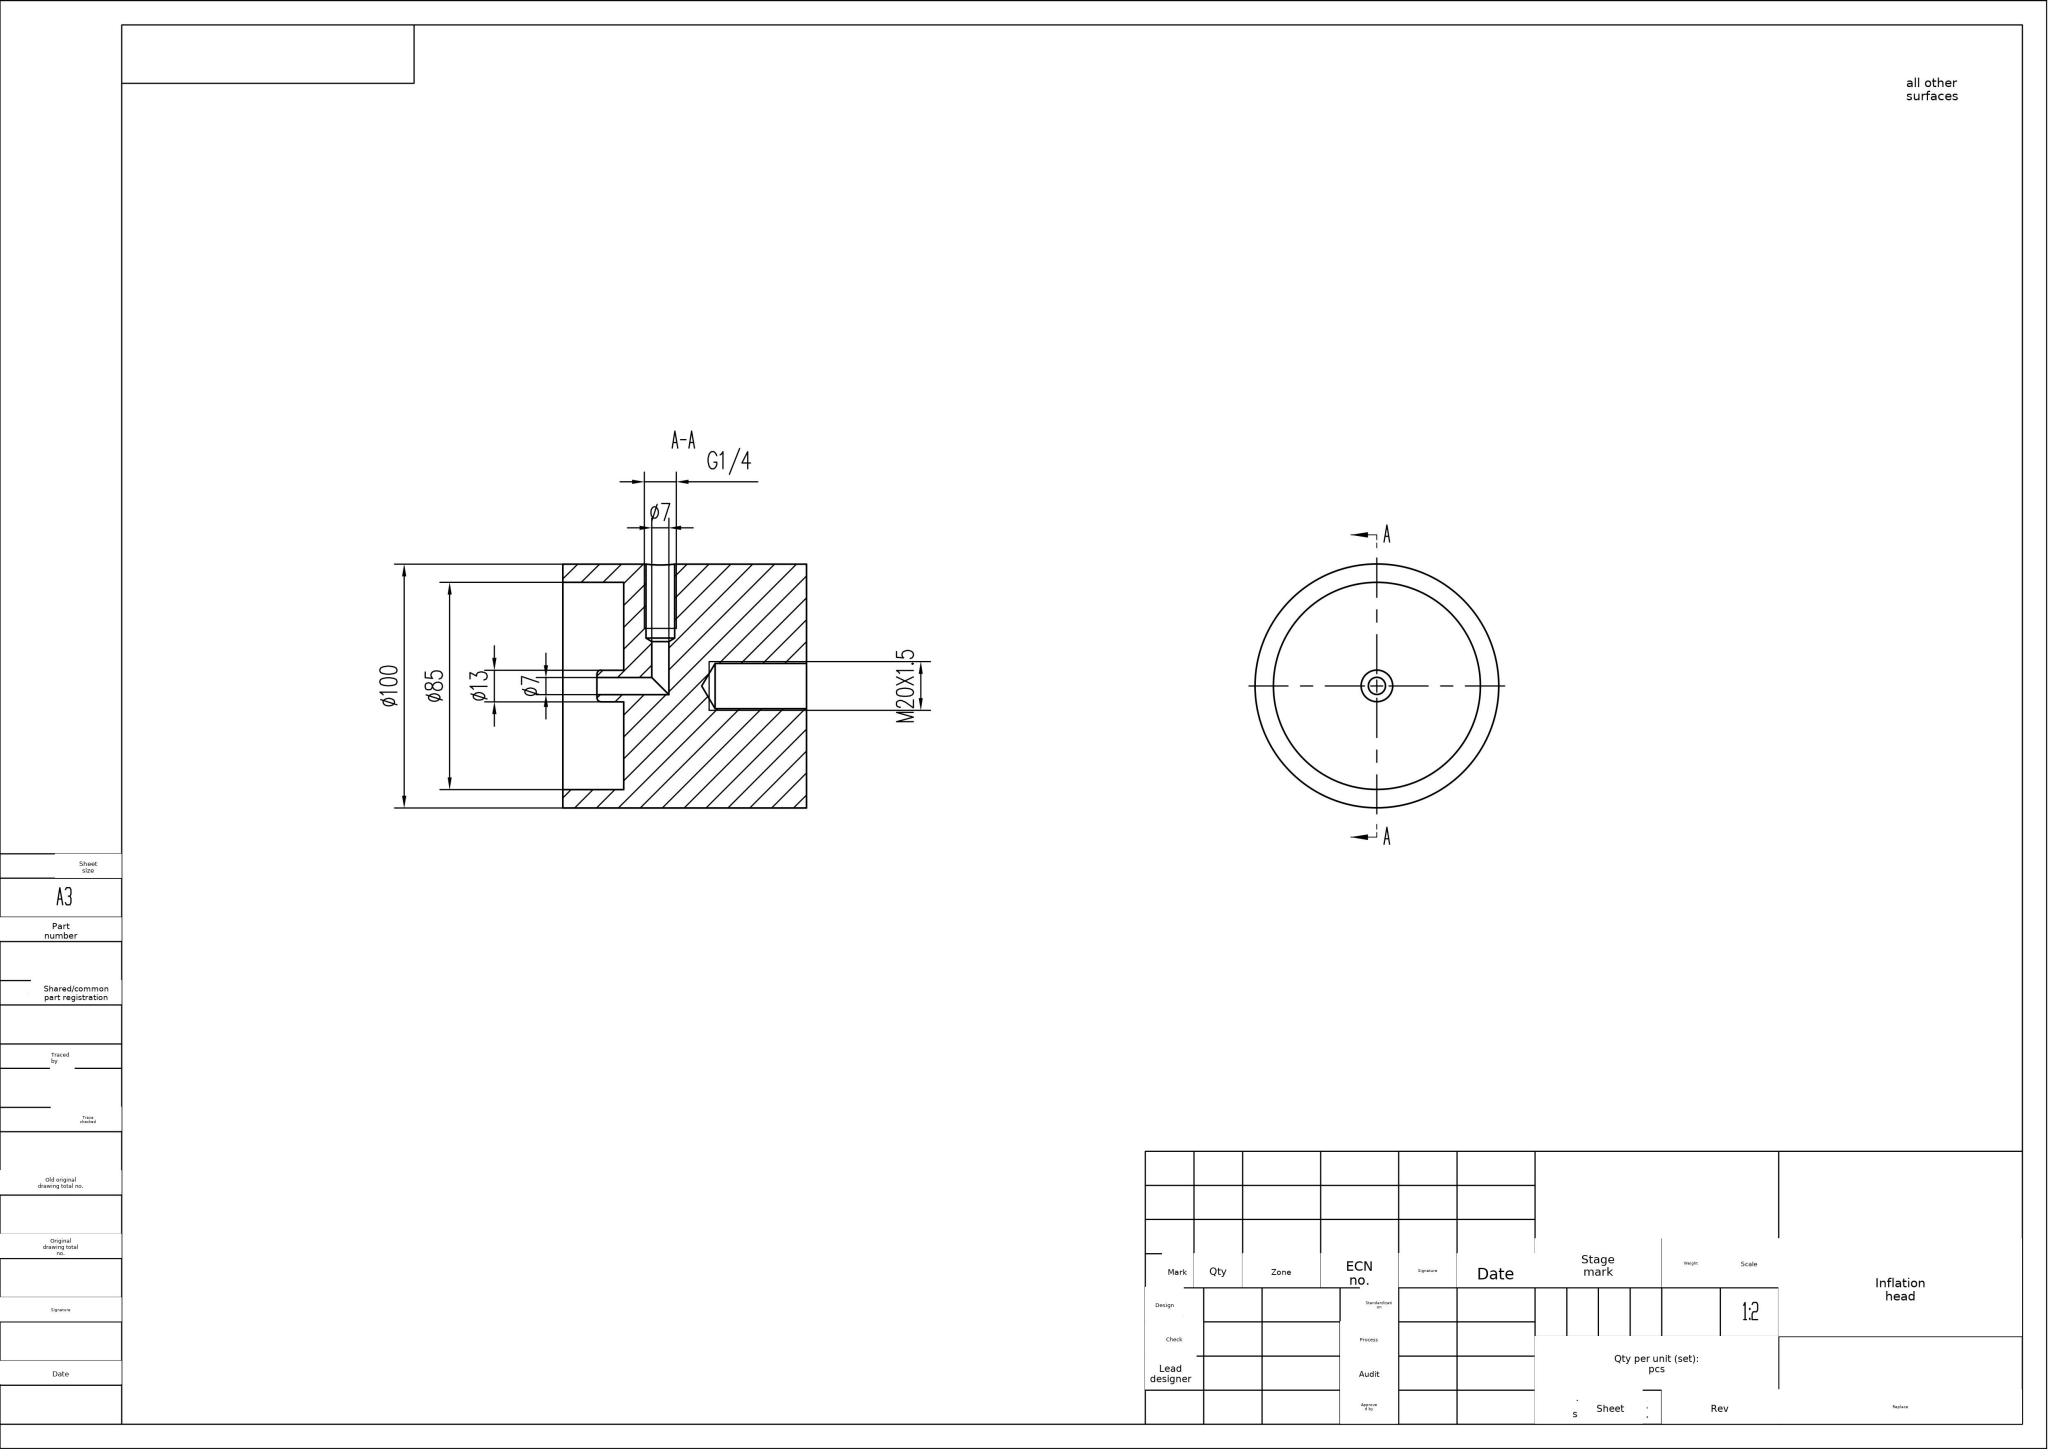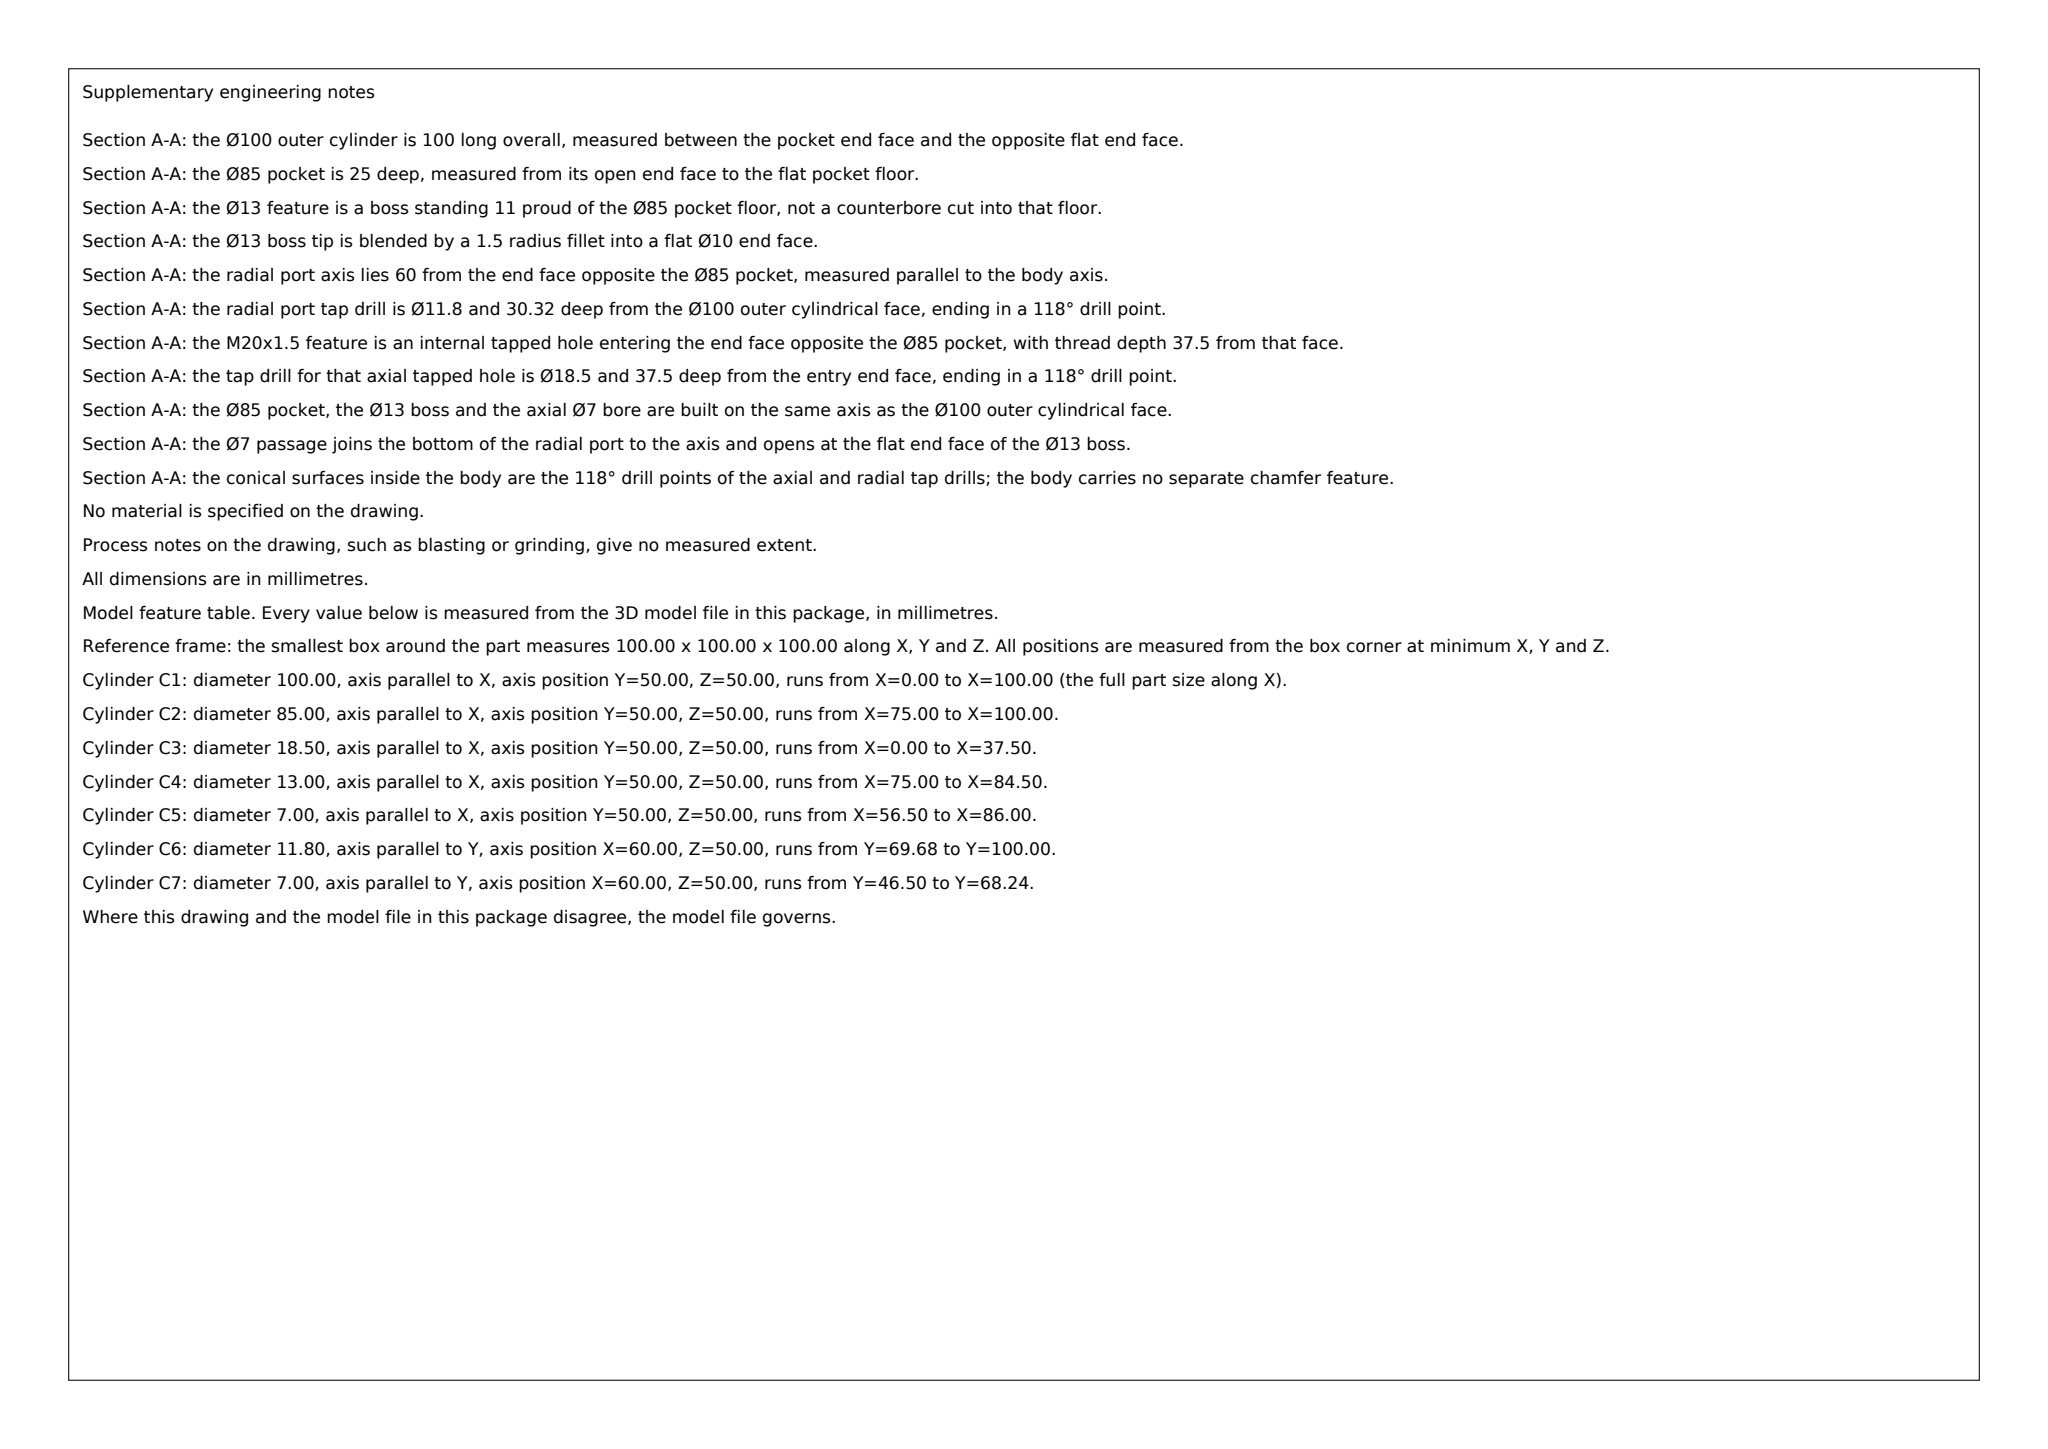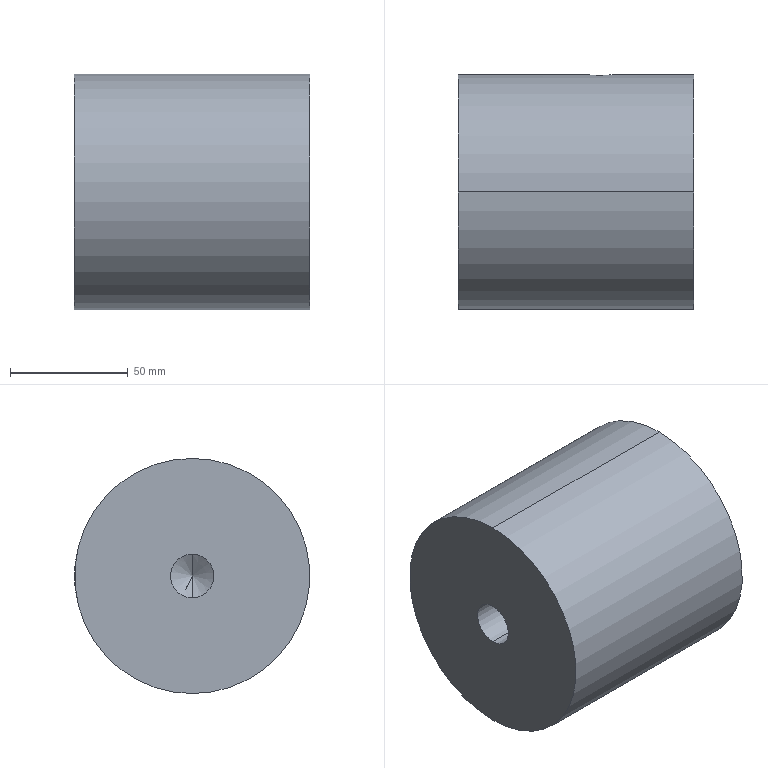Part | SolidWorks | mm | 1 solid | 24 faces | box 100 x 100 x 100 mm | volume 629288 mm3 | cylinder 14 | cone 4 | plane 4 | torus 2 | commonest cylinder face diameters 7 x4 11.8 x2 13 x2 85 x2 18.5 x2 100 x2
Drawing notes:
R1.5 FILLET AT BOT OF Ø13 BORE; ALL UNSPEC FILLETS R1.5 | from the solid: fillet_radii [[1.5,2]] at base of Ø13 x 9.5 bore (x-axis, pos 50,50)
G1/4 X-HOLE: Ø7 DP 21.74 BELOW Ø11.8 DP 30.3, INTO AXIAL Ø7 | from the solid: y-axis cyls at (x60,z50): Ø11.8 L30.32 then Ø7 L21.74 meeting Ø7 x-axis bore at y=50
build123d program:
from build123d import *

# Parameters (mm, degrees)
SKETCH1_R                  = 50
BOSS_EXTRUDE1_DEPTH        = 100
M20X1_5_TAPPED_HOLE1_D     = 18.5
M20X1_5_TAPPED_HOLE1_DEPTH = 37.5
M20X1_5_TAPPED_HOLE1_TIP   = 5.558
SKETCH5_R                  = 42.5
CUT_EXTRUDE2_DEPTH         = 25
SKETCH6_R                  = 6.5
BOSS_EXTRUDE2_DEPTH        = 11
FILLET1_R                  = 1.5
SKETCH8_R                  = 3.5
G1_4_TAPPED_HOLE1_D        = 11.8
G1_4_TAPPED_HOLE1_DEPTH    = 30.32
G1_4_TAPPED_HOLE1_TIP      = 3.545


with BuildPart() as part:
    # Sketch1 → Boss-Extrude1 (new body)
    with BuildSketch(Plane(origin=(0, 0, 0), x_dir=(0, 0, -1), z_dir=(1, 0, 0))):
        Circle(SKETCH1_R)
    extrude(amount=BOSS_EXTRUDE1_DEPTH)

    # M20x1.5 Tapped Hole1
    with Locations(Plane.ZY):
        with Locations((0, 0)):
            Hole(M20X1_5_TAPPED_HOLE1_D / 2, depth=M20X1_5_TAPPED_HOLE1_DEPTH)
            with Locations((0, 0, -(M20X1_5_TAPPED_HOLE1_DEPTH + M20X1_5_TAPPED_HOLE1_TIP / 2))):  # 118° drill point
                Cone(0, M20X1_5_TAPPED_HOLE1_D / 2, M20X1_5_TAPPED_HOLE1_TIP, mode=Mode.SUBTRACT)

    # Sketch5 → Cut-Extrude2 (cut)
    with BuildSketch(Plane(origin=(100, 0, 0), x_dir=(0, 0, -1), z_dir=(1, 0, 0))):
        Circle(SKETCH5_R)
    extrude(amount=-CUT_EXTRUDE2_DEPTH, mode=Mode.SUBTRACT)

    # Sketch6 → Boss-Extrude2 (add)
    with BuildSketch(Plane(origin=(75, 0, 0), x_dir=(0, 0, -1), z_dir=(1, 0, 0))):
        Circle(SKETCH6_R)
    extrude(amount=BOSS_EXTRUDE2_DEPTH)

    # Fillet1
    fillet1_edges = [part.edges().sort_by_distance(p)[0] for p in [
        (86, 0, 6.5),
    ]]
    fillet(fillet1_edges, radius=FILLET1_R)

    # Cut-Sweep1: sweep along a path in Sketch7
    with BuildLine(Plane.XY) as cut_sweep1_path:
        Line((60, 50), (60, 0))
        Line((60, 0), (86, 0))
    # Sketch8 → Cut-Sweep1 (sweep, cut)
    with BuildSketch(Plane(origin=(86, 0, 0), x_dir=(0, 0, -1), z_dir=(1, 0, 0))):
        Circle(SKETCH8_R)
    sweep(path=cut_sweep1_path.line, transition=Transition.RIGHT, mode=Mode.SUBTRACT)

    # G1_4 Tapped Hole1
    with Locations(Plane(origin=(0, 50, 0), x_dir=(1, 0, 0), z_dir=(0, 1, 0))):
        with Locations((60, 0)):
            Hole(G1_4_TAPPED_HOLE1_D / 2, depth=G1_4_TAPPED_HOLE1_DEPTH)
            with Locations((0, 0, -(G1_4_TAPPED_HOLE1_DEPTH + G1_4_TAPPED_HOLE1_TIP / 2))):  # 118° drill point
                Cone(0, G1_4_TAPPED_HOLE1_D / 2, G1_4_TAPPED_HOLE1_TIP, mode=Mode.SUBTRACT)


solid = part.part
STEP:
#1=CARTESIAN_POINT('',(60.,19.68,-5.9));
#2=VERTEX_POINT('',#1);
#3=CARTESIAN_POINT('',(60.,19.68,5.9));
#4=VERTEX_POINT('',#3);
#5=CARTESIAN_POINT('',(60.,19.68,0.));
#6=DIRECTION('',(-0.,1.,-0.));
#7=DIRECTION('',(0.,0.,1.));
#8=AXIS2_PLACEMENT_3D('',#5,#6,#7);
#9=CIRCLE('',#8,5.9);
#10=EDGE_CURVE('',#2,#4,#9,.T.);
#11=ORIENTED_EDGE('',*,*,#10,.F.);
#12=CARTESIAN_POINT('',(60.,49.651,-5.9));
#13=VERTEX_POINT('',#12);
#14=CARTESIAN_POINT('',(60.,50.,-5.9));
#15=DIRECTION('',(-0.,1.,-0.));
#16=VECTOR('',#15,1000.);
#17=LINE('',#14,#16);
#18=EDGE_CURVE('',#2,#13,#17,.T.);
#19=ORIENTED_EDGE('',*,*,#18,.T.);
#20=CARTESIAN_POINT('',(60.,49.651,5.9));
#21=VERTEX_POINT('',#20);
#22=CARTESIAN_POINT('',(60.,49.651,5.9));
#23=CARTESIAN_POINT('',(59.61,49.651,5.9));
#24=CARTESIAN_POINT('',(59.226,49.655,5.862));
#25=CARTESIAN_POINT('',(58.66,49.668,5.749));
#26=CARTESIAN_POINT('',(58.473,49.674,5.702));
#27=CARTESIAN_POINT('',(58.102,49.687,5.59));
#28=CARTESIAN_POINT('',(57.918,49.694,5.524));
#29=CARTESIAN_POINT('',(57.382,49.718,5.302));
#30=CARTESIAN_POINT('',(57.044,49.738,5.12));
#31=CARTESIAN_POINT('',(56.402,49.78,4.692));
#32=CARTESIAN_POINT('',(56.099,49.803,4.443));
#33=CARTESIAN_POINT('',(55.555,49.848,3.899));
#34=CARTESIAN_POINT('',(55.311,49.871,3.602));
#35=CARTESIAN_POINT('',(54.988,49.903,3.119));
#36=CARTESIAN_POINT('',(54.887,49.913,2.951));
#37=CARTESIAN_POINT('',(54.706,49.932,2.611));
#38=CARTESIAN_POINT('',(54.541,49.95,2.263));
#39=CARTESIAN_POINT('',(54.411,49.964,1.901));
#40=CARTESIAN_POINT('',(54.299,49.977,1.531));
#41=CARTESIAN_POINT('',(54.251,49.982,1.342));
#42=CARTESIAN_POINT('',(54.138,49.996,0.7704));
#43=CARTESIAN_POINT('',(54.1,50.,0.3874));
#44=CARTESIAN_POINT('',(54.1,50.,-0.383));
#45=CARTESIAN_POINT('',(54.138,49.995,-0.7743));
#46=CARTESIAN_POINT('',(54.289,49.978,-1.531));
#47=CARTESIAN_POINT('',(54.401,49.965,-1.899));
#48=CARTESIAN_POINT('',(54.623,49.941,-2.435));
#49=CARTESIAN_POINT('',(54.706,49.932,-2.612));
#50=CARTESIAN_POINT('',(54.889,49.913,-2.954));
#51=CARTESIAN_POINT('',(54.988,49.903,-3.119));
#52=CARTESIAN_POINT('',(55.308,49.871,-3.598));
#53=CARTESIAN_POINT('',(55.552,49.849,-3.896));
#54=CARTESIAN_POINT('',(56.103,49.803,-4.447));
#55=CARTESIAN_POINT('',(56.401,49.78,-4.691));
#56=CARTESIAN_POINT('',(56.88,49.748,-5.011));
#57=CARTESIAN_POINT('',(57.045,49.738,-5.11));
#58=CARTESIAN_POINT('',(57.386,49.719,-5.293));
#59=CARTESIAN_POINT('',(57.563,49.71,-5.377));
#60=CARTESIAN_POINT('',(58.099,49.686,-5.599));
#61=CARTESIAN_POINT('',(58.467,49.673,-5.71));
#62=CARTESIAN_POINT('',(59.223,49.655,-5.861));
#63=CARTESIAN_POINT('',(59.615,49.651,-5.9));
#64=CARTESIAN_POINT('',(60.,49.651,-5.9));
#65=B_SPLINE_CURVE_WITH_KNOTS('',3,(#22,#23,#24,#25,#26,#27,#28,#29,#30,#31,#32,#33,#34,#35,#36,#37,#38,#39,#40,#41,#42,#43,#44,#45,#46,#47,#48,#49,#50,#51,#52,#53,#54,#55,#56,#57,#58,#59,#60,#61,#62,#63,#64),.UNSPECIFIED.,.F.,.F.,(4,2,2,2,2,2,2,2,1,2,2,2,2,2,2,2,2,2,2,2,2,4),(0.,0.001154,0.001731,0.002308,0.003462,0.004616,0.005769,0.006346,0.006923,0.0075,0.008077,0.009231,0.01038,0.01154,0.01212,0.01269,0.01385,0.015,0.01558,0.01615,0.01731,0.01846),.UNSPECIFIED.);
#66=EDGE_CURVE('',#21,#13,#65,.T.);
#67=ORIENTED_EDGE('',*,*,#66,.F.);
#68=CARTESIAN_POINT('',(60.,50.,5.9));
#69=DIRECTION('',(-0.,1.,-0.));
#70=VECTOR('',#69,1000.);
#71=LINE('',#68,#70);
#72=EDGE_CURVE('',#4,#21,#71,.T.);
#73=ORIENTED_EDGE('',*,*,#72,.F.);
#74=EDGE_LOOP('',(#11,#19,#67,#73));
#75=FACE_OUTER_BOUND('',#74,.T.);
#76=CARTESIAN_POINT('',(60.,50.,0.));
#77=DIRECTION('',(-0.,1.,-0.));
#78=DIRECTION('',(0.,0.,1.));
#79=AXIS2_PLACEMENT_3D('',#76,#77,#78);
#80=CYLINDRICAL_SURFACE('',#79,5.9);
#81=ADVANCED_FACE('',(#75),#80,.F.);
#82=CARTESIAN_POINT('',(60.,18.238,-3.5));
#83=VERTEX_POINT('',#82);
#84=CARTESIAN_POINT('',(56.5,18.238,0.));
#85=VERTEX_POINT('',#84);
#86=CARTESIAN_POINT('',(60.,18.238,0.));
#87=DIRECTION('',(-0.,1.,-0.));
#88=DIRECTION('',(0.,0.,1.));
#89=AXIS2_PLACEMENT_3D('',#86,#87,#88);
#90=CIRCLE('',#89,3.5);
#91=EDGE_CURVE('',#83,#85,#90,.T.);
#92=ORIENTED_EDGE('',*,*,#91,.F.);
#93=CARTESIAN_POINT('',(60.,19.68,-5.9));
#94=DIRECTION('',(0.,0.515,-0.8572));
#95=VECTOR('',#94,1000.);
#96=LINE('',#93,#95);
#97=EDGE_CURVE('',#83,#2,#96,.T.);
#98=ORIENTED_EDGE('',*,*,#97,.T.);
#99=ORIENTED_EDGE('',*,*,#10,.T.);
#100=CARTESIAN_POINT('',(60.,18.238,3.5));
#101=VERTEX_POINT('',#100);
#102=CARTESIAN_POINT('',(60.,19.68,5.9));
#103=DIRECTION('',(0.,0.515,0.8572));
#104=VECTOR('',#103,1000.);
#105=LINE('',#102,#104);
#106=EDGE_CURVE('',#101,#4,#105,.T.);
#107=ORIENTED_EDGE('',*,*,#106,.F.);
#108=CARTESIAN_POINT('',(60.,18.238,0.));
#109=DIRECTION('',(-0.,1.,-0.));
#110=DIRECTION('',(0.,0.,1.));
#111=AXIS2_PLACEMENT_3D('',#108,#109,#110);
#112=CIRCLE('',#111,3.5);
#113=EDGE_CURVE('',#85,#101,#112,.T.);
#114=ORIENTED_EDGE('',*,*,#113,.F.);
#115=EDGE_LOOP('',(#92,#98,#99,#107,#114));
#116=FACE_OUTER_BOUND('',#115,.T.);
#117=CARTESIAN_POINT('',(60.,19.68,0.));
#118=DIRECTION('',(-0.,1.,-0.));
#119=DIRECTION('',(0.,0.,1.));
#120=AXIS2_PLACEMENT_3D('',#117,#118,#119);
#121=CONICAL_SURFACE('',#120,5.9,1.03);
#122=ADVANCED_FACE('',(#116),#121,.F.);
#123=CARTESIAN_POINT('',(63.5,18.238,0.));
#124=VERTEX_POINT('',#123);
#125=CARTESIAN_POINT('',(60.,18.238,0.));
#126=DIRECTION('',(-0.,1.,-0.));
#127=DIRECTION('',(0.,0.,1.));
#128=AXIS2_PLACEMENT_3D('',#125,#126,#127);
#129=CIRCLE('',#128,3.5);
#130=EDGE_CURVE('',#124,#83,#129,.T.);
#131=ORIENTED_EDGE('',*,*,#130,.T.);
#132=ORIENTED_EDGE('',*,*,#91,.T.);
#133=CARTESIAN_POINT('',(56.5,-3.5,0.));
#134=VERTEX_POINT('',#133);
#135=CARTESIAN_POINT('',(56.5,51.,0.));
#136=DIRECTION('',(0.,-1.,0.));
#137=VECTOR('',#136,1000.);
#138=LINE('',#135,#137);
#139=EDGE_CURVE('',#85,#134,#138,.T.);
#140=ORIENTED_EDGE('',*,*,#139,.T.);
#141=CARTESIAN_POINT('',(60.,0.,-3.5));
#142=VERTEX_POINT('',#141);
#143=CARTESIAN_POINT('',(60.,0.,-3.5));
#144=CARTESIAN_POINT('',(57.95,-2.05,-3.5));
#145=CARTESIAN_POINT('',(56.5,-3.5,-2.05));
#146=CARTESIAN_POINT('',(56.5,-3.5,0.));
#147=(BOUNDED_CURVE()B_SPLINE_CURVE(3,(#143,#144,#145,#146),.UNSPECIFIED.,.F.,.T.)B_SPLINE_CURVE_WITH_KNOTS((4,4),(4.712,6.283),.UNSPECIFIED.)CURVE()GEOMETRIC_REPRESENTATION_ITEM()RATIONAL_B_SPLINE_CURVE((1.,0.8047,0.8047,1.))REPRESENTATION_ITEM(''));
#148=EDGE_CURVE('',#142,#134,#147,.T.);
#149=ORIENTED_EDGE('',*,*,#148,.F.);
#150=CARTESIAN_POINT('',(63.5,3.5,0.));
#151=VERTEX_POINT('',#150);
#152=CARTESIAN_POINT('',(63.5,3.5,0.));
#153=CARTESIAN_POINT('',(63.5,3.5,-2.05));
#154=CARTESIAN_POINT('',(62.05,2.05,-3.5));
#155=CARTESIAN_POINT('',(60.,0.,-3.5));
#156=(BOUNDED_CURVE()B_SPLINE_CURVE(3,(#152,#153,#154,#155),.UNSPECIFIED.,.F.,.F.)B_SPLINE_CURVE_WITH_KNOTS((4,4),(3.142,4.712),.UNSPECIFIED.)CURVE()GEOMETRIC_REPRESENTATION_ITEM()RATIONAL_B_SPLINE_CURVE((1.,0.8047,0.8047,1.))REPRESENTATION_ITEM(''));
#157=EDGE_CURVE('',#151,#142,#156,.T.);
#158=ORIENTED_EDGE('',*,*,#157,.F.);
#159=CARTESIAN_POINT('',(63.5,51.,0.));
#160=DIRECTION('',(0.,-1.,0.));
#161=VECTOR('',#160,1000.);
#162=LINE('',#159,#161);
#163=EDGE_CURVE('',#124,#151,#162,.T.);
#164=ORIENTED_EDGE('',*,*,#163,.F.);
#165=EDGE_LOOP('',(#131,#132,#140,#149,#158,#164));
#166=FACE_OUTER_BOUND('',#165,.T.);
#167=CARTESIAN_POINT('',(60.,51.,0.));
#168=DIRECTION('',(0.,-1.,0.));
#169=DIRECTION('',(1.,0.,0.));
#170=AXIS2_PLACEMENT_3D('',#167,#168,#169);
#171=CYLINDRICAL_SURFACE('',#170,3.5);
#172=ADVANCED_FACE('',(#166),#171,.F.);
#173=ORIENTED_EDGE('',*,*,#148,.T.);
#174=CARTESIAN_POINT('',(60.,0.,3.5));
#175=VERTEX_POINT('',#174);
#176=CARTESIAN_POINT('',(56.5,-3.5,0.));
#177=CARTESIAN_POINT('',(56.5,-3.5,2.05));
#178=CARTESIAN_POINT('',(57.95,-2.05,3.5));
#179=CARTESIAN_POINT('',(60.,0.,3.5));
#180=(BOUNDED_CURVE()B_SPLINE_CURVE(3,(#176,#177,#178,#179),.UNSPECIFIED.,.F.,.F.)B_SPLINE_CURVE_WITH_KNOTS((4,4),(0.,1.571),.UNSPECIFIED.)CURVE()GEOMETRIC_REPRESENTATION_ITEM()RATIONAL_B_SPLINE_CURVE((1.,0.8047,0.8047,1.))REPRESENTATION_ITEM(''));
#181=EDGE_CURVE('',#134,#175,#180,.T.);
#182=ORIENTED_EDGE('',*,*,#181,.T.);
#183=CARTESIAN_POINT('',(86.,0.,3.5));
#184=VERTEX_POINT('',#183);
#185=CARTESIAN_POINT('',(52.2,0.,3.5));
#186=DIRECTION('',(1.,0.,0.));
#187=VECTOR('',#186,1000.);
#188=LINE('',#185,#187);
#189=EDGE_CURVE('',#175,#184,#188,.T.);
#190=ORIENTED_EDGE('',*,*,#189,.T.);
#191=CARTESIAN_POINT('',(86.,0.,-3.5));
#192=VERTEX_POINT('',#191);
#193=CARTESIAN_POINT('',(86.,0.,0.));
#194=DIRECTION('',(-1.,-0.,-0.));
#195=DIRECTION('',(0.,0.,-1.));
#196=AXIS2_PLACEMENT_3D('',#193,#194,#195);
#197=CIRCLE('',#196,3.5);
#198=EDGE_CURVE('',#192,#184,#197,.T.);
#199=ORIENTED_EDGE('',*,*,#198,.F.);
#200=CARTESIAN_POINT('',(52.2,0.,-3.5));
#201=DIRECTION('',(1.,0.,0.));
#202=VECTOR('',#201,1000.);
#203=LINE('',#200,#202);
#204=EDGE_CURVE('',#142,#192,#203,.T.);
#205=ORIENTED_EDGE('',*,*,#204,.F.);
#206=EDGE_LOOP('',(#173,#182,#190,#199,#205));
#207=FACE_OUTER_BOUND('',#206,.T.);
#208=CARTESIAN_POINT('',(52.2,0.,0.));
#209=DIRECTION('',(1.,0.,0.));
#210=DIRECTION('',(0.,0.,-1.));
#211=AXIS2_PLACEMENT_3D('',#208,#209,#210);
#212=CYLINDRICAL_SURFACE('',#211,3.5);
#213=ADVANCED_FACE('',(#207),#212,.F.);
#214=CARTESIAN_POINT('',(84.5,-0.,6.5));
#215=VERTEX_POINT('',#214);
#216=CARTESIAN_POINT('',(84.5,0.,-6.5));
#217=VERTEX_POINT('',#216);
#218=CARTESIAN_POINT('',(84.5,0.,0.));
#219=DIRECTION('',(-1.,-0.,-0.));
#220=DIRECTION('',(0.,0.,-1.));
#221=AXIS2_PLACEMENT_3D('',#218,#219,#220);
#222=CIRCLE('',#221,6.5);
#223=EDGE_CURVE('',#215,#217,#222,.T.);
#224=ORIENTED_EDGE('',*,*,#223,.F.);
#225=CARTESIAN_POINT('',(86.,0.,5.));
#226=VERTEX_POINT('',#225);
#227=CARTESIAN_POINT('',(84.5,0.,5.));
#228=DIRECTION('',(-0.,1.,-0.));
#229=DIRECTION('',(0.,0.,1.));
#230=AXIS2_PLACEMENT_3D('',#227,#228,#229);
#231=CIRCLE('',#230,1.5);
#232=EDGE_CURVE('',#215,#226,#231,.T.);
#233=ORIENTED_EDGE('',*,*,#232,.T.);
#234=CARTESIAN_POINT('',(86.,0.,-5.));
#235=VERTEX_POINT('',#234);
#236=CARTESIAN_POINT('',(86.,0.,0.));
#237=DIRECTION('',(1.,0.,0.));
#238=DIRECTION('',(0.,0.,-1.));
#239=AXIS2_PLACEMENT_3D('',#236,#237,#238);
#240=CIRCLE('',#239,5.);
#241=EDGE_CURVE('',#235,#226,#240,.T.);
#242=ORIENTED_EDGE('',*,*,#241,.F.);
#243=CARTESIAN_POINT('',(84.5,0.,-5.));
#244=DIRECTION('',(0.,-1.,-0.));
#245=DIRECTION('',(0.,0.,-1.));
#246=AXIS2_PLACEMENT_3D('',#243,#244,#245);
#247=CIRCLE('',#246,1.5);
#248=EDGE_CURVE('',#217,#235,#247,.T.);
#249=ORIENTED_EDGE('',*,*,#248,.F.);
#250=EDGE_LOOP('',(#224,#233,#242,#249));
#251=FACE_OUTER_BOUND('',#250,.T.);
#252=CARTESIAN_POINT('',(84.5,0.,0.));
#253=DIRECTION('',(1.,0.,0.));
#254=DIRECTION('',(0.,0.,-1.));
#255=AXIS2_PLACEMENT_3D('',#252,#253,#254);
#256=TOROIDAL_SURFACE('',#255,5.,1.5);
#257=ADVANCED_FACE('',(#251),#256,.T.);
#258=ORIENTED_EDGE('',*,*,#223,.T.);
#259=CARTESIAN_POINT('',(75.,0.,-6.5));
#260=VERTEX_POINT('',#259);
#261=CARTESIAN_POINT('',(86.,0.,-6.5));
#262=DIRECTION('',(-1.,-0.,-0.));
#263=VECTOR('',#262,1000.);
#264=LINE('',#261,#263);
#265=EDGE_CURVE('',#217,#260,#264,.T.);
#266=ORIENTED_EDGE('',*,*,#265,.T.);
#267=CARTESIAN_POINT('',(75.,-0.,6.5));
#268=VERTEX_POINT('',#267);
#269=CARTESIAN_POINT('',(75.,0.,0.));
#270=DIRECTION('',(1.,0.,0.));
#271=DIRECTION('',(0.,0.,-1.));
#272=AXIS2_PLACEMENT_3D('',#269,#270,#271);
#273=CIRCLE('',#272,6.5);
#274=EDGE_CURVE('',#260,#268,#273,.T.);
#275=ORIENTED_EDGE('',*,*,#274,.T.);
#276=CARTESIAN_POINT('',(86.,-0.,6.5));
#277=DIRECTION('',(-1.,-0.,-0.));
#278=VECTOR('',#277,1000.);
#279=LINE('',#276,#278);
#280=EDGE_CURVE('',#215,#268,#279,.T.);
#281=ORIENTED_EDGE('',*,*,#280,.F.);
#282=EDGE_LOOP('',(#258,#266,#275,#281));
#283=FACE_OUTER_BOUND('',#282,.T.);
#284=CARTESIAN_POINT('',(86.,0.,0.));
#285=DIRECTION('',(-1.,-0.,-0.));
#286=DIRECTION('',(0.,-0.,1.));
#287=AXIS2_PLACEMENT_3D('',#284,#285,#286);
#288=CYLINDRICAL_SURFACE('',#287,6.5);
#289=ADVANCED_FACE('',(#283),#288,.T.);
#290=CARTESIAN_POINT('',(75.,0.,42.5));
#291=VERTEX_POINT('',#290);
#292=CARTESIAN_POINT('',(75.,0.,-42.5));
#293=VERTEX_POINT('',#292);
#294=CARTESIAN_POINT('',(75.,0.,0.));
#295=DIRECTION('',(1.,0.,0.));
#296=DIRECTION('',(0.,0.,-1.));
#297=AXIS2_PLACEMENT_3D('',#294,#295,#296);
#298=CIRCLE('',#297,42.5);
#299=EDGE_CURVE('',#291,#293,#298,.T.);
#300=ORIENTED_EDGE('',*,*,#299,.F.);
#301=CARTESIAN_POINT('',(100.,0.,42.5));
#302=VERTEX_POINT('',#301);
#303=CARTESIAN_POINT('',(75.,0.,42.5));
#304=DIRECTION('',(1.,0.,0.));
#305=VECTOR('',#304,1000.);
#306=LINE('',#303,#305);
#307=EDGE_CURVE('',#291,#302,#306,.T.);
#308=ORIENTED_EDGE('',*,*,#307,.T.);
#309=CARTESIAN_POINT('',(100.,0.,-42.5));
#310=VERTEX_POINT('',#309);
#311=CARTESIAN_POINT('',(100.,0.,0.));
#312=DIRECTION('',(1.,0.,0.));
#313=DIRECTION('',(0.,0.,-1.));
#314=AXIS2_PLACEMENT_3D('',#311,#312,#313);
#315=CIRCLE('',#314,42.5);
#316=EDGE_CURVE('',#302,#310,#315,.T.);
#317=ORIENTED_EDGE('',*,*,#316,.T.);
#318=CARTESIAN_POINT('',(75.,0.,-42.5));
#319=DIRECTION('',(1.,0.,0.));
#320=VECTOR('',#319,1000.);
#321=LINE('',#318,#320);
#322=EDGE_CURVE('',#293,#310,#321,.T.);
#323=ORIENTED_EDGE('',*,*,#322,.F.);
#324=EDGE_LOOP('',(#300,#308,#317,#323));
#325=FACE_OUTER_BOUND('',#324,.T.);
#326=CARTESIAN_POINT('',(75.,0.,0.));
#327=DIRECTION('',(1.,0.,0.));
#328=DIRECTION('',(0.,0.,-1.));
#329=AXIS2_PLACEMENT_3D('',#326,#327,#328);
#330=CYLINDRICAL_SURFACE('',#329,42.5);
#331=ADVANCED_FACE('',(#325),#330,.F.);
#332=CARTESIAN_POINT('',(37.5,0.,-9.25));
#333=VERTEX_POINT('',#332);
#334=CARTESIAN_POINT('',(37.5,-0.,9.25));
#335=VERTEX_POINT('',#334);
#336=CARTESIAN_POINT('',(37.5,0.,0.));
#337=DIRECTION('',(-1.,-0.,-0.));
#338=DIRECTION('',(0.,-0.,1.));
#339=AXIS2_PLACEMENT_3D('',#336,#337,#338);
#340=CIRCLE('',#339,9.25);
#341=EDGE_CURVE('',#333,#335,#340,.T.);
#342=ORIENTED_EDGE('',*,*,#341,.F.);
#343=CARTESIAN_POINT('',(0.,0.,-9.25));
#344=VERTEX_POINT('',#343);
#345=CARTESIAN_POINT('',(-0.,0.,-9.25));
#346=DIRECTION('',(-1.,-0.,-0.));
#347=VECTOR('',#346,1000.);
#348=LINE('',#345,#347);
#349=EDGE_CURVE('',#333,#344,#348,.T.);
#350=ORIENTED_EDGE('',*,*,#349,.T.);
#351=CARTESIAN_POINT('',(0.,-0.,9.25));
#352=VERTEX_POINT('',#351);
#353=CARTESIAN_POINT('',(0.,0.,0.));
#354=DIRECTION('',(-1.,-0.,-0.));
#355=DIRECTION('',(0.,-0.,1.));
#356=AXIS2_PLACEMENT_3D('',#353,#354,#355);
#357=CIRCLE('',#356,9.25);
#358=EDGE_CURVE('',#344,#352,#357,.T.);
#359=ORIENTED_EDGE('',*,*,#358,.T.);
#360=CARTESIAN_POINT('',(0.,-0.,9.25));
#361=DIRECTION('',(-1.,-0.,-0.));
#362=VECTOR('',#361,1000.);
#363=LINE('',#360,#362);
#364=EDGE_CURVE('',#335,#352,#363,.T.);
#365=ORIENTED_EDGE('',*,*,#364,.F.);
#366=EDGE_LOOP('',(#342,#350,#359,#365));
#367=FACE_OUTER_BOUND('',#366,.T.);
#368=CARTESIAN_POINT('',(0.,0.,0.));
#369=DIRECTION('',(-1.,-0.,-0.));
#370=DIRECTION('',(0.,-0.,1.));
#371=AXIS2_PLACEMENT_3D('',#368,#369,#370);
#372=CYLINDRICAL_SURFACE('',#371,9.25);
#373=ADVANCED_FACE('',(#367),#372,.F.);
#374=CARTESIAN_POINT('',(43.058,0.,0.));
#375=VERTEX_POINT('',#374);
#376=CARTESIAN_POINT('',(37.5,-0.,9.25));
#377=DIRECTION('',(-0.515,-0.,0.8572));
#378=VECTOR('',#377,1000.);
#379=LINE('',#376,#378);
#380=EDGE_CURVE('',#375,#335,#379,.T.);
#381=ORIENTED_EDGE('',*,*,#380,.F.);
#382=CARTESIAN_POINT('',(37.5,0.,-9.25));
#383=DIRECTION('',(-0.515,0.,-0.8572));
#384=VECTOR('',#383,1000.);
#385=LINE('',#382,#384);
#386=EDGE_CURVE('',#375,#333,#385,.T.);
#387=ORIENTED_EDGE('',*,*,#386,.T.);
#388=ORIENTED_EDGE('',*,*,#341,.T.);
#389=EDGE_LOOP('',(#381,#387,#388));
#390=FACE_OUTER_BOUND('',#389,.T.);
#391=CARTESIAN_POINT('',(37.5,0.,0.));
#392=DIRECTION('',(-1.,-0.,-0.));
#393=DIRECTION('',(0.,-0.,1.));
#394=AXIS2_PLACEMENT_3D('',#391,#392,#393);
#395=CONICAL_SURFACE('',#394,9.25,1.03);
#396=ADVANCED_FACE('',(#390),#395,.F.);
#397=ORIENTED_EDGE('',*,*,#66,.T.);
#398=CARTESIAN_POINT('',(60.,49.651,-5.9));
#399=CARTESIAN_POINT('',(60.385,49.651,-5.9));
#400=CARTESIAN_POINT('',(60.768,49.655,-5.863));
#401=CARTESIAN_POINT('',(61.339,49.668,-5.749));
#402=CARTESIAN_POINT('',(61.529,49.674,-5.702));
#403=CARTESIAN_POINT('',(61.898,49.687,-5.59));
#404=CARTESIAN_POINT('',(62.261,49.701,-5.46));
#405=CARTESIAN_POINT('',(62.609,49.719,-5.296));
#406=CARTESIAN_POINT('',(62.949,49.738,-5.114));
#407=CARTESIAN_POINT('',(63.117,49.748,-5.013));
#408=CARTESIAN_POINT('',(63.6,49.78,-4.69));
#409=CARTESIAN_POINT('',(63.897,49.803,-4.446));
#410=CARTESIAN_POINT('',(64.441,49.848,-3.903));
#411=CARTESIAN_POINT('',(64.69,49.871,-3.6));
#412=CARTESIAN_POINT('',(65.119,49.913,-2.959));
#413=CARTESIAN_POINT('',(65.3,49.933,-2.621));
#414=CARTESIAN_POINT('',(65.523,49.957,-2.085));
#415=CARTESIAN_POINT('',(65.589,49.964,-1.901));
#416=CARTESIAN_POINT('',(65.701,49.977,-1.53));
#417=CARTESIAN_POINT('',(65.748,49.982,-1.343));
#418=CARTESIAN_POINT('',(65.861,49.995,-0.7778));
#419=CARTESIAN_POINT('',(65.9,50.,-0.3944));
#420=CARTESIAN_POINT('',(65.9,50.,0.3858));
#421=CARTESIAN_POINT('',(65.862,49.996,0.7694));
#422=CARTESIAN_POINT('',(65.75,49.983,1.335));
#423=CARTESIAN_POINT('',(65.704,49.977,1.522));
#424=CARTESIAN_POINT('',(65.591,49.964,1.893));
#425=CARTESIAN_POINT('',(65.526,49.957,2.077));
#426=CARTESIAN_POINT('',(65.304,49.933,2.613));
#427=CARTESIAN_POINT('',(65.123,49.914,2.952));
#428=CARTESIAN_POINT('',(64.695,49.872,3.594));
#429=CARTESIAN_POINT('',(64.446,49.849,3.897));
#430=CARTESIAN_POINT('',(63.903,49.803,4.441));
#431=CARTESIAN_POINT('',(63.607,49.78,4.685));
#432=CARTESIAN_POINT('',(63.123,49.749,5.009));
#433=CARTESIAN_POINT('',(62.956,49.738,5.11));
#434=CARTESIAN_POINT('',(62.616,49.719,5.292));
#435=CARTESIAN_POINT('',(62.442,49.71,5.374));
#436=CARTESIAN_POINT('',(61.91,49.686,5.595));
#437=CARTESIAN_POINT('',(61.538,49.673,5.709));
#438=CARTESIAN_POINT('',(60.776,49.655,5.862));
#439=CARTESIAN_POINT('',(60.39,49.651,5.9));
#440=CARTESIAN_POINT('',(60.,49.651,5.9));
#441=B_SPLINE_CURVE_WITH_KNOTS('',3,(#398,#399,#400,#401,#402,#403,#404,#405,#406,#407,#408,#409,#410,#411,#412,#413,#414,#415,#416,#417,#418,#419,#420,#421,#422,#423,#424,#425,#426,#427,#428,#429,#430,#431,#432,#433,#434,#435,#436,#437,#438,#439,#440),.UNSPECIFIED.,.F.,.F.,(4,2,2,1,2,2,2,2,2,2,2,2,2,2,2,2,2,2,2,2,2,4),(0.01846,0.01962,0.02019,0.02077,0.02135,0.02192,0.02308,0.02423,0.02538,0.02596,0.02654,0.02769,0.02884,0.02942,0.03,0.03115,0.03231,0.03346,0.03404,0.03461,0.03577,0.03692),.UNSPECIFIED.);
#442=EDGE_CURVE('',#13,#21,#441,.T.);
#443=ORIENTED_EDGE('',*,*,#442,.T.);
#444=EDGE_LOOP('',(#397,#443));
#445=FACE_BOUND('',#444,.T.);
#446=CARTESIAN_POINT('',(100.,0.,-50.));
#447=VERTEX_POINT('',#446);
#448=CARTESIAN_POINT('',(100.,-0.,50.));
#449=VERTEX_POINT('',#448);
#450=CARTESIAN_POINT('',(100.,0.,0.));
#451=DIRECTION('',(1.,0.,0.));
#452=DIRECTION('',(0.,0.,-1.));
#453=AXIS2_PLACEMENT_3D('',#450,#451,#452);
#454=CIRCLE('',#453,50.);
#455=EDGE_CURVE('',#447,#449,#454,.T.);
#456=ORIENTED_EDGE('',*,*,#455,.F.);
#457=CARTESIAN_POINT('',(0.,0.,-50.));
#458=VERTEX_POINT('',#457);
#459=CARTESIAN_POINT('',(100.,0.,-50.));
#460=DIRECTION('',(-1.,-0.,-0.));
#461=VECTOR('',#460,1000.);
#462=LINE('',#459,#461);
#463=EDGE_CURVE('',#447,#458,#462,.T.);
#464=ORIENTED_EDGE('',*,*,#463,.T.);
#465=CARTESIAN_POINT('',(-0.,-0.,50.));
#466=VERTEX_POINT('',#465);
#467=CARTESIAN_POINT('',(0.,0.,0.));
#468=DIRECTION('',(1.,0.,0.));
#469=DIRECTION('',(-0.,0.,-1.));
#470=AXIS2_PLACEMENT_3D('',#467,#468,#469);
#471=CIRCLE('',#470,50.);
#472=EDGE_CURVE('',#458,#466,#471,.T.);
#473=ORIENTED_EDGE('',*,*,#472,.T.);
#474=CARTESIAN_POINT('',(100.,-0.,50.));
#475=DIRECTION('',(-1.,-0.,-0.));
#476=VECTOR('',#475,1000.);
#477=LINE('',#474,#476);
#478=EDGE_CURVE('',#449,#466,#477,.T.);
#479=ORIENTED_EDGE('',*,*,#478,.F.);
#480=EDGE_LOOP('',(#456,#464,#473,#479));
#481=FACE_OUTER_BOUND('',#480,.T.);
#482=CARTESIAN_POINT('',(100.,0.,0.));
#483=DIRECTION('',(-1.,-0.,-0.));
#484=DIRECTION('',(0.,-0.,1.));
#485=AXIS2_PLACEMENT_3D('',#482,#483,#484);
#486=CYLINDRICAL_SURFACE('',#485,50.);
#487=ADVANCED_FACE('',(#445,#481),#486,.T.);
#488=ORIENTED_EDGE('',*,*,#463,.F.);
#489=CARTESIAN_POINT('',(100.,0.,0.));
#490=DIRECTION('',(1.,0.,0.));
#491=DIRECTION('',(0.,0.,-1.));
#492=AXIS2_PLACEMENT_3D('',#489,#490,#491);
#493=CIRCLE('',#492,50.);
#494=EDGE_CURVE('',#449,#447,#493,.T.);
#495=ORIENTED_EDGE('',*,*,#494,.F.);
#496=ORIENTED_EDGE('',*,*,#478,.T.);
#497=CARTESIAN_POINT('',(0.,0.,0.));
#498=DIRECTION('',(1.,0.,0.));
#499=DIRECTION('',(-0.,0.,-1.));
#500=AXIS2_PLACEMENT_3D('',#497,#498,#499);
#501=CIRCLE('',#500,50.);
#502=EDGE_CURVE('',#466,#458,#501,.T.);
#503=ORIENTED_EDGE('',*,*,#502,.T.);
#504=EDGE_LOOP('',(#488,#495,#496,#503));
#505=FACE_OUTER_BOUND('',#504,.T.);
#506=CARTESIAN_POINT('',(100.,0.,0.));
#507=DIRECTION('',(-1.,-0.,-0.));
#508=DIRECTION('',(0.,-0.,1.));
#509=AXIS2_PLACEMENT_3D('',#506,#507,#508);
#510=CYLINDRICAL_SURFACE('',#509,50.);
#511=ADVANCED_FACE('',(#505),#510,.T.);
#512=CARTESIAN_POINT('',(100.,0.,0.));
#513=DIRECTION('',(1.,0.,0.));
#514=DIRECTION('',(0.,0.,-1.));
#515=AXIS2_PLACEMENT_3D('',#512,#513,#514);
#516=CIRCLE('',#515,42.5);
#517=EDGE_CURVE('',#310,#302,#516,.T.);
#518=ORIENTED_EDGE('',*,*,#517,.F.);
#519=ORIENTED_EDGE('',*,*,#316,.F.);
#520=EDGE_LOOP('',(#518,#519));
#521=FACE_BOUND('',#520,.T.);
#522=ORIENTED_EDGE('',*,*,#494,.T.);
#523=ORIENTED_EDGE('',*,*,#455,.T.);
#524=EDGE_LOOP('',(#522,#523));
#525=FACE_OUTER_BOUND('',#524,.T.);
#526=CARTESIAN_POINT('',(100.,0.,0.));
#527=DIRECTION('',(1.,0.,-0.));
#528=DIRECTION('',(-0.,0.,-1.));
#529=AXIS2_PLACEMENT_3D('',#526,#527,#528);
#530=PLANE('',#529);
#531=ADVANCED_FACE('',(#521,#525),#530,.T.);
#532=CARTESIAN_POINT('',(0.,0.,0.));
#533=DIRECTION('',(-1.,-0.,-0.));
#534=DIRECTION('',(0.,-0.,1.));
#535=AXIS2_PLACEMENT_3D('',#532,#533,#534);
#536=CIRCLE('',#535,9.25);
#537=EDGE_CURVE('',#352,#344,#536,.T.);
#538=ORIENTED_EDGE('',*,*,#537,.F.);
#539=ORIENTED_EDGE('',*,*,#358,.F.);
#540=EDGE_LOOP('',(#538,#539));
#541=FACE_BOUND('',#540,.T.);
#542=ORIENTED_EDGE('',*,*,#502,.F.);
#543=ORIENTED_EDGE('',*,*,#472,.F.);
#544=EDGE_LOOP('',(#542,#543));
#545=FACE_OUTER_BOUND('',#544,.T.);
#546=CARTESIAN_POINT('',(0.,0.,0.));
#547=DIRECTION('',(1.,0.,-0.));
#548=DIRECTION('',(-0.,0.,-1.));
#549=AXIS2_PLACEMENT_3D('',#546,#547,#548);
#550=PLANE('',#549);
#551=ADVANCED_FACE('',(#541,#545),#550,.F.);
#552=ORIENTED_EDGE('',*,*,#386,.F.);
#553=ORIENTED_EDGE('',*,*,#380,.T.);
#554=CARTESIAN_POINT('',(37.5,0.,0.));
#555=DIRECTION('',(-1.,-0.,-0.));
#556=DIRECTION('',(0.,-0.,1.));
#557=AXIS2_PLACEMENT_3D('',#554,#555,#556);
#558=CIRCLE('',#557,9.25);
#559=EDGE_CURVE('',#335,#333,#558,.T.);
#560=ORIENTED_EDGE('',*,*,#559,.T.);
#561=EDGE_LOOP('',(#552,#553,#560));
#562=FACE_OUTER_BOUND('',#561,.T.);
#563=CARTESIAN_POINT('',(37.5,0.,0.));
#564=DIRECTION('',(-1.,-0.,-0.));
#565=DIRECTION('',(0.,-0.,1.));
#566=AXIS2_PLACEMENT_3D('',#563,#564,#565);
#567=CONICAL_SURFACE('',#566,9.25,1.03);
#568=ADVANCED_FACE('',(#562),#567,.F.);
#569=ORIENTED_EDGE('',*,*,#349,.F.);
#570=ORIENTED_EDGE('',*,*,#559,.F.);
#571=ORIENTED_EDGE('',*,*,#364,.T.);
#572=ORIENTED_EDGE('',*,*,#537,.T.);
#573=EDGE_LOOP('',(#569,#570,#571,#572));
#574=FACE_OUTER_BOUND('',#573,.T.);
#575=CARTESIAN_POINT('',(0.,0.,0.));
#576=DIRECTION('',(-1.,-0.,-0.));
#577=DIRECTION('',(0.,-0.,1.));
#578=AXIS2_PLACEMENT_3D('',#575,#576,#577);
#579=CYLINDRICAL_SURFACE('',#578,9.25);
#580=ADVANCED_FACE('',(#574),#579,.F.);
#581=ORIENTED_EDGE('',*,*,#307,.F.);
#582=CARTESIAN_POINT('',(75.,0.,0.));
#583=DIRECTION('',(1.,0.,0.));
#584=DIRECTION('',(0.,0.,-1.));
#585=AXIS2_PLACEMENT_3D('',#582,#583,#584);
#586=CIRCLE('',#585,42.5);
#587=EDGE_CURVE('',#293,#291,#586,.T.);
#588=ORIENTED_EDGE('',*,*,#587,.F.);
#589=ORIENTED_EDGE('',*,*,#322,.T.);
#590=ORIENTED_EDGE('',*,*,#517,.T.);
#591=EDGE_LOOP('',(#581,#588,#589,#590));
#592=FACE_OUTER_BOUND('',#591,.T.);
#593=CARTESIAN_POINT('',(75.,0.,0.));
#594=DIRECTION('',(1.,0.,0.));
#595=DIRECTION('',(0.,0.,-1.));
#596=AXIS2_PLACEMENT_3D('',#593,#594,#595);
#597=CYLINDRICAL_SURFACE('',#596,42.5);
#598=ADVANCED_FACE('',(#592),#597,.F.);
#599=CARTESIAN_POINT('',(75.,0.,0.));
#600=DIRECTION('',(1.,0.,0.));
#601=DIRECTION('',(0.,0.,-1.));
#602=AXIS2_PLACEMENT_3D('',#599,#600,#601);
#603=CIRCLE('',#602,6.5);
#604=EDGE_CURVE('',#268,#260,#603,.T.);
#605=ORIENTED_EDGE('',*,*,#604,.F.);
#606=ORIENTED_EDGE('',*,*,#274,.F.);
#607=EDGE_LOOP('',(#605,#606));
#608=FACE_BOUND('',#607,.T.);
#609=ORIENTED_EDGE('',*,*,#587,.T.);
#610=ORIENTED_EDGE('',*,*,#299,.T.);
#611=EDGE_LOOP('',(#609,#610));
#612=FACE_OUTER_BOUND('',#611,.T.);
#613=CARTESIAN_POINT('',(75.,0.,0.));
#614=DIRECTION('',(1.,0.,-0.));
#615=DIRECTION('',(-0.,0.,-1.));
#616=AXIS2_PLACEMENT_3D('',#613,#614,#615);
#617=PLANE('',#616);
#618=ADVANCED_FACE('',(#608,#612),#617,.T.);
#619=ORIENTED_EDGE('',*,*,#265,.F.);
#620=CARTESIAN_POINT('',(84.5,0.,0.));
#621=DIRECTION('',(-1.,-0.,-0.));
#622=DIRECTION('',(0.,0.,-1.));
#623=AXIS2_PLACEMENT_3D('',#620,#621,#622);
#624=CIRCLE('',#623,6.5);
#625=EDGE_CURVE('',#217,#215,#624,.T.);
#626=ORIENTED_EDGE('',*,*,#625,.T.);
#627=ORIENTED_EDGE('',*,*,#280,.T.);
#628=ORIENTED_EDGE('',*,*,#604,.T.);
#629=EDGE_LOOP('',(#619,#626,#627,#628));
#630=FACE_OUTER_BOUND('',#629,.T.);
#631=CARTESIAN_POINT('',(86.,0.,0.));
#632=DIRECTION('',(-1.,-0.,-0.));
#633=DIRECTION('',(0.,-0.,1.));
#634=AXIS2_PLACEMENT_3D('',#631,#632,#633);
#635=CYLINDRICAL_SURFACE('',#634,6.5);
#636=ADVANCED_FACE('',(#630),#635,.T.);
#637=ORIENTED_EDGE('',*,*,#198,.T.);
#638=CARTESIAN_POINT('',(86.,0.,0.));
#639=DIRECTION('',(-1.,-0.,-0.));
#640=DIRECTION('',(0.,0.,-1.));
#641=AXIS2_PLACEMENT_3D('',#638,#639,#640);
#642=CIRCLE('',#641,3.5);
#643=EDGE_CURVE('',#184,#192,#642,.T.);
#644=ORIENTED_EDGE('',*,*,#643,.T.);
#645=EDGE_LOOP('',(#637,#644));
#646=FACE_BOUND('',#645,.T.);
#647=ORIENTED_EDGE('',*,*,#241,.T.);
#648=CARTESIAN_POINT('',(86.,0.,0.));
#649=DIRECTION('',(1.,0.,0.));
#650=DIRECTION('',(0.,0.,-1.));
#651=AXIS2_PLACEMENT_3D('',#648,#649,#650);
#652=CIRCLE('',#651,5.);
#653=EDGE_CURVE('',#226,#235,#652,.T.);
#654=ORIENTED_EDGE('',*,*,#653,.T.);
#655=EDGE_LOOP('',(#647,#654));
#656=FACE_OUTER_BOUND('',#655,.T.);
#657=CARTESIAN_POINT('',(86.,0.,0.));
#658=DIRECTION('',(1.,0.,-0.));
#659=DIRECTION('',(-0.,0.,-1.));
#660=AXIS2_PLACEMENT_3D('',#657,#658,#659);
#661=PLANE('',#660);
#662=ADVANCED_FACE('',(#646,#656),#661,.T.);
#663=ORIENTED_EDGE('',*,*,#232,.F.);
#664=ORIENTED_EDGE('',*,*,#625,.F.);
#665=ORIENTED_EDGE('',*,*,#248,.T.);
#666=ORIENTED_EDGE('',*,*,#653,.F.);
#667=EDGE_LOOP('',(#663,#664,#665,#666));
#668=FACE_OUTER_BOUND('',#667,.T.);
#669=CARTESIAN_POINT('',(84.5,0.,0.));
#670=DIRECTION('',(1.,0.,0.));
#671=DIRECTION('',(0.,0.,-1.));
#672=AXIS2_PLACEMENT_3D('',#669,#670,#671);
#673=TOROIDAL_SURFACE('',#672,5.,1.5);
#674=ADVANCED_FACE('',(#668),#673,.T.);
#675=ORIENTED_EDGE('',*,*,#189,.F.);
#676=CARTESIAN_POINT('',(60.,0.,3.5));
#677=CARTESIAN_POINT('',(62.05,2.05,3.5));
#678=CARTESIAN_POINT('',(63.5,3.5,2.05));
#679=CARTESIAN_POINT('',(63.5,3.5,0.));
#680=(BOUNDED_CURVE()B_SPLINE_CURVE(3,(#676,#677,#678,#679),.UNSPECIFIED.,.F.,.T.)B_SPLINE_CURVE_WITH_KNOTS((4,4),(1.571,3.142),.UNSPECIFIED.)CURVE()GEOMETRIC_REPRESENTATION_ITEM()RATIONAL_B_SPLINE_CURVE((1.,0.8047,0.8047,1.))REPRESENTATION_ITEM(''));
#681=EDGE_CURVE('',#175,#151,#680,.T.);
#682=ORIENTED_EDGE('',*,*,#681,.T.);
#683=ORIENTED_EDGE('',*,*,#157,.T.);
#684=ORIENTED_EDGE('',*,*,#204,.T.);
#685=ORIENTED_EDGE('',*,*,#643,.F.);
#686=EDGE_LOOP('',(#675,#682,#683,#684,#685));
#687=FACE_OUTER_BOUND('',#686,.T.);
#688=CARTESIAN_POINT('',(52.2,0.,0.));
#689=DIRECTION('',(1.,0.,0.));
#690=DIRECTION('',(0.,0.,-1.));
#691=AXIS2_PLACEMENT_3D('',#688,#689,#690);
#692=CYLINDRICAL_SURFACE('',#691,3.5);
#693=ADVANCED_FACE('',(#687),#692,.F.);
#694=ORIENTED_EDGE('',*,*,#139,.F.);
#695=ORIENTED_EDGE('',*,*,#113,.T.);
#696=CARTESIAN_POINT('',(60.,18.238,0.));
#697=DIRECTION('',(-0.,1.,-0.));
#698=DIRECTION('',(0.,0.,1.));
#699=AXIS2_PLACEMENT_3D('',#696,#697,#698);
#700=CIRCLE('',#699,3.5);
#701=EDGE_CURVE('',#101,#124,#700,.T.);
#702=ORIENTED_EDGE('',*,*,#701,.T.);
#703=ORIENTED_EDGE('',*,*,#163,.T.);
#704=ORIENTED_EDGE('',*,*,#681,.F.);
#705=ORIENTED_EDGE('',*,*,#181,.F.);
#706=EDGE_LOOP('',(#694,#695,#702,#703,#704,#705));
#707=FACE_OUTER_BOUND('',#706,.T.);
#708=CARTESIAN_POINT('',(60.,51.,0.));
#709=DIRECTION('',(0.,-1.,0.));
#710=DIRECTION('',(1.,0.,0.));
#711=AXIS2_PLACEMENT_3D('',#708,#709,#710);
#712=CYLINDRICAL_SURFACE('',#711,3.5);
#713=ADVANCED_FACE('',(#707),#712,.F.);
#714=ORIENTED_EDGE('',*,*,#97,.F.);
#715=ORIENTED_EDGE('',*,*,#130,.F.);
#716=ORIENTED_EDGE('',*,*,#701,.F.);
#717=ORIENTED_EDGE('',*,*,#106,.T.);
#718=CARTESIAN_POINT('',(60.,19.68,0.));
#719=DIRECTION('',(-0.,1.,-0.));
#720=DIRECTION('',(0.,0.,1.));
#721=AXIS2_PLACEMENT_3D('',#718,#719,#720);
#722=CIRCLE('',#721,5.9);
#723=EDGE_CURVE('',#4,#2,#722,.T.);
#724=ORIENTED_EDGE('',*,*,#723,.T.);
#725=EDGE_LOOP('',(#714,#715,#716,#717,#724));
#726=FACE_OUTER_BOUND('',#725,.T.);
#727=CARTESIAN_POINT('',(60.,19.68,0.));
#728=DIRECTION('',(-0.,1.,-0.));
#729=DIRECTION('',(0.,0.,1.));
#730=AXIS2_PLACEMENT_3D('',#727,#728,#729);
#731=CONICAL_SURFACE('',#730,5.9,1.03);
#732=ADVANCED_FACE('',(#726),#731,.F.);
#733=ORIENTED_EDGE('',*,*,#18,.F.);
#734=ORIENTED_EDGE('',*,*,#723,.F.);
#735=ORIENTED_EDGE('',*,*,#72,.T.);
#736=ORIENTED_EDGE('',*,*,#442,.F.);
#737=EDGE_LOOP('',(#733,#734,#735,#736));
#738=FACE_OUTER_BOUND('',#737,.T.);
#739=CARTESIAN_POINT('',(60.,50.,0.));
#740=DIRECTION('',(-0.,1.,-0.));
#741=DIRECTION('',(0.,0.,1.));
#742=AXIS2_PLACEMENT_3D('',#739,#740,#741);
#743=CYLINDRICAL_SURFACE('',#742,5.9);
#744=ADVANCED_FACE('',(#738),#743,.F.);
#745=CLOSED_SHELL('',(#81,#122,#172,#213,#257,#289,#331,#373,#396,#487,#511,#531,#551,#568,#580,#598,#618,#636,#662,#674,#693,#713,#732,#744));
#746=MANIFOLD_SOLID_BREP('',#745);
#747=CARTESIAN_POINT('',(0.,0.,0.));
#748=DIRECTION('',(0.,0.,1.));
#749=DIRECTION('',(1.,0.,0.));
#750=AXIS2_PLACEMENT_3D('',#747,#748,#749);
#751=(LENGTH_UNIT()NAMED_UNIT(*)SI_UNIT(.MILLI.,.METRE.));
#752=UNCERTAINTY_MEASURE_WITH_UNIT(LENGTH_MEASURE(0.00001),#751,'','');
#753=(NAMED_UNIT(*)PLANE_ANGLE_UNIT()SI_UNIT($,.RADIAN.));
#754=(NAMED_UNIT(*)SI_UNIT($,.STERADIAN.)SOLID_ANGLE_UNIT());
#755=(GEOMETRIC_REPRESENTATION_CONTEXT(3)GLOBAL_UNCERTAINTY_ASSIGNED_CONTEXT((#752))GLOBAL_UNIT_ASSIGNED_CONTEXT((#751,#753,#754))REPRESENTATION_CONTEXT('',''));
#756=ADVANCED_BREP_SHAPE_REPRESENTATION('',(#746,#750),#755);